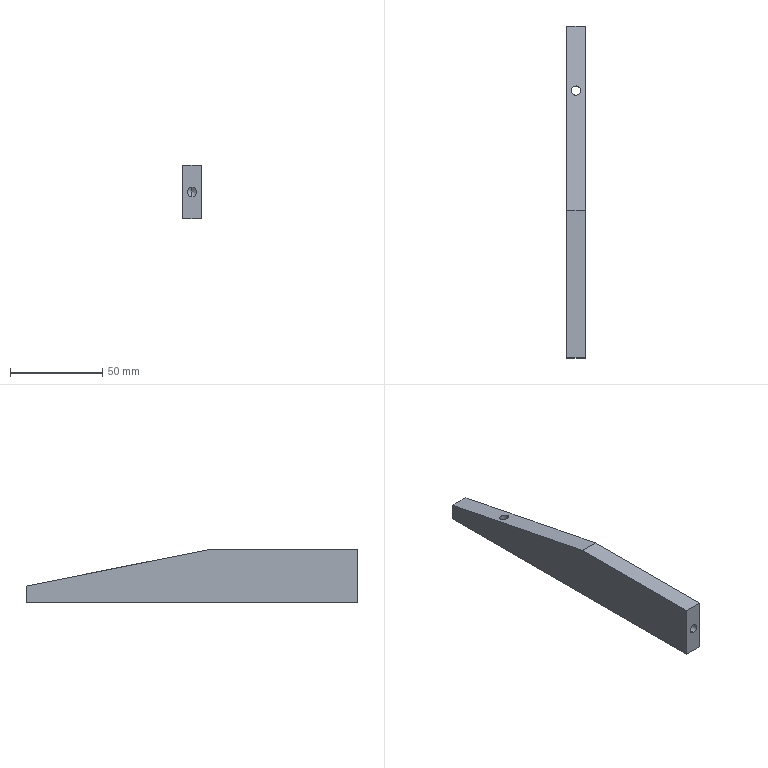Component | SolidWorks | ReinforcingRib9.26-1 | 1 solid | 25 faces | box 10 x 180 x 29 mm | volume 40433 mm3 | cylinder 10 | cone 8 | plane 7 | commonest cylinder face diameters 5 x10
build123d program:
from build123d import *

# Parameters (mm, degrees)
SKETCH1_W             = 10
SKETCH1_H             = 180
BOSS_EXTRUDE1_DEPTH   = 29
CHAMFER1_SIZE         = 20
CHAMFER1_SIZE2        = 100
M6_TAPPED_HOLE1_D     = 5
M6_TAPPED_HOLE1_DEPTH = 18
M6_TAPPED_HOLE1_TIP   = 1.502
LPATTERN1_COUNT       = 4
LPATTERN1_PITCH       = 40


with BuildPart() as part:
    # Sketch1 → Boss-Extrude1 (new body)
    with BuildSketch(Plane.XY):
        with Locations((5, -90)):
            Rectangle(SKETCH1_W, SKETCH1_H)
    extrude(amount=BOSS_EXTRUDE1_DEPTH)

    # Chamfer1
    chamfer1_edges = [part.edges().sort_by_distance(p)[0] for p in [
        (5, 0, 29),
    ]]
    chamfer1_side = [part.faces().sort_by_distance(p)[0] for p in [
        (5, 0, 14.5),
    ]]
    chamfer(chamfer1_edges, length=CHAMFER1_SIZE, length2=CHAMFER1_SIZE2, reference=chamfer1_side[0])

    # M6 Tapped Hole1
    with Locations(Plane.XZ.offset(180)):
        with Locations((5, 14.5)):
            Hole(M6_TAPPED_HOLE1_D / 2, depth=M6_TAPPED_HOLE1_DEPTH)
            with Locations((0, 0, -(M6_TAPPED_HOLE1_DEPTH + M6_TAPPED_HOLE1_TIP / 2))):  # 118° drill point
                Cone(0, M6_TAPPED_HOLE1_D / 2, M6_TAPPED_HOLE1_TIP, mode=Mode.SUBTRACT)

    # Sketch6 → M6 Tapped Hole2 (revolve, cut)
    with BuildSketch(Plane(origin=(5, -155, 0), x_dir=(0, 1, 0), z_dir=(1, 0, 0))):
        Polygon((0, 0), (0, 19.502), (2.5, 18), (2.5, 0), align=None)
    m6_tapped_hole2 = revolve(axis=Axis((5, -155, -6.35), (0, 0, 1)), mode=Mode.SUBTRACT)

    # LPattern1: M6 Tapped Hole2 ×4
    with Locations(*[(0, i * LPATTERN1_PITCH, 0) for i in range(1, LPATTERN1_COUNT)]):
        add(m6_tapped_hole2, mode=Mode.SUBTRACT)


solid = part.part

# Placed as in the assembly
solid = solid.moved(Location((251, 17, 40.5), (0, 0, 0)))